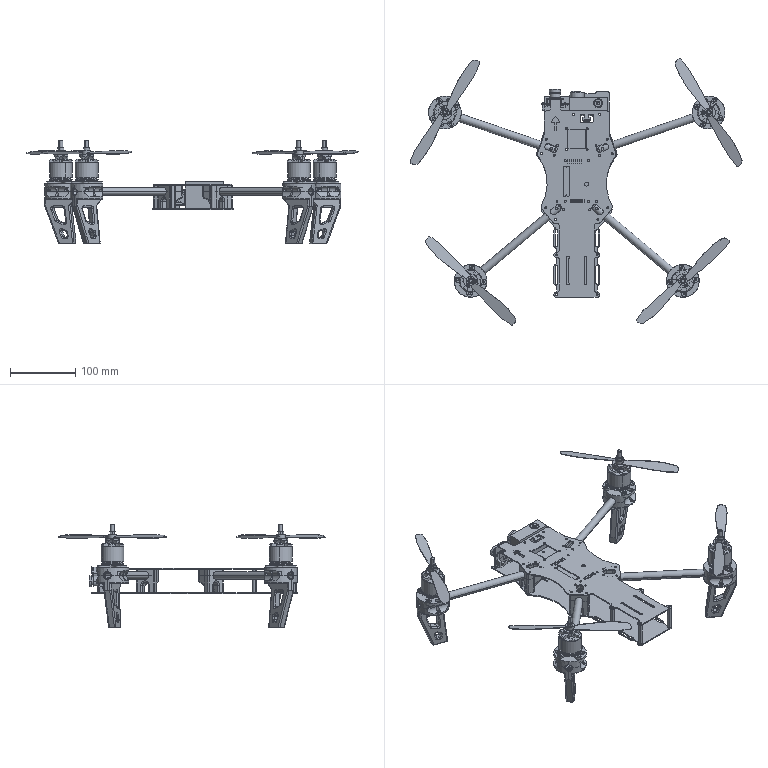Assembly | SolidWorks | mm | 49 component files | 49 solids | 2994 faces | box 508.26 x 408.35 x 158.75 mm | volume 593246 mm3 | cylinder 1614 | plane 994 | cone 152 | torus 112 | spline 76 | sphere 46 | commonest cylinder face diameters 4 x487 3 x165 8 x126 35 x76 2 x74 2.5 x64 16 x60 30 x48
Bill of materials:
Actuator | 1 |  | Thin rectangular plate with four corner holes. A stepped cylindrical body sticks out from one face, and several small rectangular blocks sit on the plate. Overall it resembles a board-mounted camera/lens module.
Adjuster | 4 |  | Short thick-walled cylindrical ring/bushing with a through bore. The outer edge on one end is chamfered or conical.
BaseConnectionPart | 4 |  | Flat, thin four-armed cross/X-shaped plate with rounded arm ends, generous fillets between arms, and a central hole. Each arm has two through-holes.
Camera | 1 |  | Rectangular block with a short cylindrical boss on one face. A shallow circular feature (ring or button outline) is on the top face.
ConnectingRod | 4 |  | Long straight hollow round tube with small radial cross-holes near each end.
Connector | 4 |  | Round disc base with a central upright cylindrical pin that has a chamfered tip. The disc has three through-holes with counterbores. The underside has large curved scallop cuts.
FanBlade | 4 |  | Two-bladed propeller-like part. A small cylindrical hub with a central through-bore has two long, thin, tapered and twisted blades sticking out in opposite directions.
LowerPartOfBracket | 4 |  | Short cylindrical puck-shaped hub. The top face has a small central hole, four radial slots and two counterbored holes. Large arched cutouts are around the lower side wall.
LowerPlate | 1 |  | Long, very thin, flat plate with a complex outline. It has a narrow waist with large concave curved sides and a central round hole. It also has many small holes, long slots, a T/key-shaped cutout, and paired slots along the edges of one end.
Motor | 4 |  | Cylindrical can-shaped body that resembles an outrunner-style motor. The top has spoked openings, a raised central boss, and small holes. Grooves and flange steps are near the bottom, and a short shaft sticks out at each end.
SupportPlate | 1 |  | Thin rectangular plate with a large central circular hole. There are small rectangular tabs on one short edge and matching notches on the opposite edge, with rounded corners.
UpperAndLowerPlateConnection | 4 |  | Thick, roughly square block with rounded corners and notched edges. It has a central elongated (obround) through-opening and four corner through-holes. A semicircular saddle cut runs across the underside.
UpperAndLowerPlateLowerConnectionPart | 4 |  | Block-shaped part with a semicircular channel running across its top face. Two flat flanges sit on either side of the channel, each with two through holes, so there are four holes in total. Underneath are two legs with an arched opening between them, which forms a channel at right angles to the top one.
UpperAndLowerPlateSupportColumn | 4 |  | Straight hollow cylinder (a tube or spacer) with a single concentric through bore and plain flat ends.
UpperPartOfBracket | 4 |  | Round flat-topped head on a tapered, slanted arm that gets narrower toward its free end. The top of the head has a wide central groove with a smaller hole in its floor. It also has two through holes, a small dome-shaped bump and several smaller grooves running parallel to the main one. The arm is a web with stiffening edges and two lightening cutouts with rounded corners: a large trapezoid and a smaller rounded slot.
UpperPlate | 1 |  | Thin flat plate, long and roughly symmetrical about its long axis. It has a wider middle section with curved, waisted sides and a narrower rectangular tail with two long parallel slots. A small tab sticks out from one end. The plate has many small round holes, four angled oblong slots, a square cutout, a long central slot, a single larger hole, two patches of tiny holes in a grid, an arrow-shaped cutout and a squared C-shaped cutout.
Mates:
1. concentric | LowerPlate-1 face at (-71.048, 32.401, 1000) dir (0, 0, 1) r 1.5 | UpperAndLowerPlateLowerConnectionPart-1 face at (-71.048, 32.401, 1027.6) dir (0, 0, -1) r 1.5
2. concentric | LowerPlate-1 face at (-63.432, 54.633, 1000) dir (0, 0, 1) r 1.5 | UpperAndLowerPlateLowerConnectionPart-1 face at (-63.432, 54.633, 1027.6) dir (0, 0, -1) r 1.5
3. coincident | LowerPlate-1 face at (14.261, -183.575, 1001.6) dir (0, 0, 1) | UpperAndLowerPlateLowerConnectionPart-1 face at (-50.912, 29.468, 1001.6) dir (0, 0, -1)
4. concentric | UpperAndLowerPlateLowerConnectionPart-1 face at (-71.048, 32.401, 1027.6) dir (0, 0, -1) r 1.5 | UpperAndLowerPlateConnection-1 face at (-71.048, 32.401, 1037.6) dir (0, 0, -1) r 1.5
5. concentric | UpperAndLowerPlateLowerConnectionPart-1 face at (-46.2, 44.766, 1027.6) dir (0, 0, -1) r 1.5 | UpperAndLowerPlateConnection-1 face at (-46.2, 44.766, 1037.6) dir (0, 0, -1) r 1.5
6. coincident | UpperAndLowerPlateLowerConnectionPart-1 face at (-50.912, 29.468, 1027.6) dir (0, 0, 1) | UpperAndLowerPlateConnection-1 face at (-59.183, 54.499, 1027.6) dir (0, 0, -1)
7. concentric | UpperAndLowerPlateLowerConnectionPart-1 face at (-44.535, 35.74, 1027.6) dir (-0.946, 0.3241, 0) r 6 | ConnectingRod-1 face at (-51.158, 38.008, 1027.6) dir (-0.946, 0.3241, 0) r 6
8. concentric | UpperAndLowerPlateConnection-1 face at (-70.078, 44.49, 1032.6) dir (0, 0, 1) r 2 | ConnectingRod-1 face at (-70.078, 44.49, 1033.6) dir (0, 0, -1) r 2
9. concentric | ConnectingRod-1 face at (-51.158, 38.008, 1027.6) dir (-0.946, 0.3241, 0) r 6 | LowerPartOfBracket-1 face at (-194.955, 87.266, 1027.6) dir (-0.946, 0.3241, 0) r 6
10. concentric | ConnectingRod-1 face at (-235.635, 101.2, 1033.6) dir (0, 0, -1) r 2 | LowerPartOfBracket-1 face at (-235.635, 101.2, 1032.6) dir (0, 0, 1) r 2
11. concentric | ConnectingRod-1 face at (-51.158, 38.008, 1027.6) dir (-0.946, 0.3241, 0) r 6 | UpperPartOfBracket-1 face at (-194.955, 87.266, 1027.6) dir (-0.946, 0.3241, 0) r 6
12. coincident | UpperPartOfBracket-1 face at (-218.606, 95.367, 1027.6) dir (0, 0, 1) | LowerPartOfBracket-1 face at (-218.606, 95.367, 1027.6) dir (0, 0, -1)
13. concentric | ConnectingRod-1 face at (-235.635, 101.2, 1033.6) dir (0, 0, -1) r 2 | UpperPartOfBracket-1 face at (-235.635, 101.2, 1022.6) dir (0, 0, -1) r 2
14. width | BaseConnectionPart-1 face at (-216.847, 91.775, 1042.6) dir (0.4398, -0.8981, 0) | BaseConnectionPart-1 face at (-220.365, 98.96, 1042.6) dir (-0.4398, 0.8981, 0) | LowerPartOfBracket-1 face at (-224.911, 90.053, 1026.263) dir (-0.4398, 0.8981, 0) | LowerPartOfBracket-1 face at (-226.67, 93.645, 1026.263) dir (0.4398, -0.8981, 0)
15. width | BaseConnectionPart-1 face at (-222.198, 93.608, 1042.6) dir (-0.8981, -0.4398, 0) | BaseConnectionPart-1 face at (-215.014, 97.126, 1042.6) dir (0.8981, 0.4398, 0) | LowerPartOfBracket-1 face at (-223.921, 101.672, 1026.263) dir (0.8981, 0.4398, 0) | LowerPartOfBracket-1 face at (-220.328, 103.431, 1026.263) dir (-0.8981, -0.4398, 0)
16. coincident | LowerPartOfBracket-1 face at (-218.606, 95.367, 1039.6) dir (0, 0, 1) | BaseConnectionPart-1 face at (-218.606, 95.367, 1039.6) dir (0, 0, -1)
17. concentric | BaseConnectionPart-1 face at (-213.108, 84.141, 1039.6) dir (0, 0, -1) r 1.7 | Motor-1 face at (-213.108, 84.141, 1042.6) dir (0, 0, -1) r 1.25
18. concentric | BaseConnectionPart-1 face at (-210.074, 99.545, 1039.6) dir (0, 0, -1) r 1.7 | Motor-1 face at (-210.074, 99.545, 1042.6) dir (0, 0, -1) r 1.25
19. concentric | BaseConnectionPart-1 face at (-218.606, 95.367, 1039.6) dir (0, 0, 1) r 2.25 | Motor-1 face at (-218.606, 95.367, 1078.15) dir (0, 0, 1) r 2
20. coincident | BaseConnectionPart-1 face at (-218.606, 95.367, 1042.6) dir (0, 0, 1) | Motor-1 face at (-220.402, 94.488, 1042.6) dir (0, 0, -1)
21. concentric | Motor-1 face at (-222.79, 89.143, 1069.85) dir (0, 0, 1) r 1 | Connector-1 face at (-222.79, 89.143, 1084.35) dir (0, 0, 1) r 1.45
22. concentric | Motor-1 face at (-211.123, 94.856, 1069.85) dir (0, 0, 1) r 1 | Connector-1 face at (-211.123, 94.856, 1084.35) dir (0, 0, 1) r 1.45
23. coincident | Motor-1 face at (-223.096, 93.168, 1078.35) dir (0, 0, 1) | Connector-1 face at (-218.606, 95.367, 1078.35) dir (0, 0, -1)
24. concentric | Connector-1 face at (-218.606, 95.367, 1076.35) dir (0, 0, -1) r 3 | FanBlade-1 face at (-218.606, 95.367, 1075.65) dir (0, 0, 1) r 3.25
25. coincident | Connector-1 face at (-209.892, 89.509, 1084.35) dir (0, 0, 1) | FanBlade-1 face at (-218.606, 95.367, 1084.35) dir (0, 0, -1)
26. coincident | LowerPlate-1 face at (14.261, -183.575, 1001.6) dir (0, 0, 1) | SupportPlate-1 face at (-47.616, 116.675, 1001.6) dir (0, 0, -1)
27. parallel | LowerPlate-1 face at (33.261, 120.425, 1001.6) dir (0, 1, 0) | SupportPlate-1 face at (-50.116, 116.675, 1018.85) dir (0, 1, 0)
28. parallel | LowerPlate-1 face at (-66.739, 64.711, 1001.6) dir (-1, 0, 0) | SupportPlate-1 face at (-62.616, 116.675, 1000.1) dir (-1, 0, 0)
29. coincident | LowerPlate-1 face at (-61.077, 116.675, 1000) dir (0, -1, 0) | SupportPlate-1 face at (-50.116, 116.675, 1018.85) dir (0, 1, 0)
30. lock | LowerPlate-1 reference at (0, 0, 0) dir (1, 0, 0) | SupportPlate-1 reference at (0, 0, 0) dir (1, 0, 0)
31. concentric | SupportPlate-1 face at (-50.116, 116.675, 1018.85) dir (0, -1, 0) r 8 | Actuator-1 face at (-50.116, 108.825, 1018.85) dir (0, -1, 0) r 8
32. coincident | SupportPlate-1 face at (-50.116, 115.175, 1018.85) dir (0, -1, 0) | Actuator-1 face at (-50.116, 115.175, 1018.85) dir (0, 1, 0)
33. parallel | SupportPlate-1 face at (-54.616, 116.675, 1037.6) dir (0, 0, 1) | Actuator-1 face at (-70.116, 107.325, 1031.35) dir (0, 0, 1)
34. coincident | LowerPlate-1 face at (14.261, -183.575, 1001.6) dir (0, 0, 1) | Camera-1 face at (30.917, 118.685, 1001.6) dir (0, 0, -1)
35. parallel | LowerPlate-1 face at (-51.739, -165.575, 1001.6) dir (-1, 0, 0) | UpperPlate-3 face at (-43.739, -176.647, 1039.2) dir (-1, 0, 0)
36. concentric | LowerPlate-1 face at (-47.739, -183.575, 1000) dir (0, 0, 1) r 1.5 | UpperPlate-3 face at (-47.739, -183.575, 1037.6) dir (0, 0, 1) r 1.5
37. concentric | UpperAndLowerPlateSupportColumn-1 face at (-47.739, -122.575, 1037.6) dir (0, 0, -1) r 1.5 | UpperPlate-3 face at (-47.739, -122.575, 1037.6) dir (0, 0, 1) r 1.5
38. coincident | LowerPlate-1 face at (14.261, -183.575, 1001.6) dir (0, 0, 1) | UpperAndLowerPlateSupportColumn-1 face at (-47.739, -122.575, 1001.6) dir (0, 0, -1)
39. concentric | UpperPlate-3 face at (-47.739, -183.575, 1037.6) dir (0, 0, 1) r 1.5 | UpperAndLowerPlateSupportColumn-2 face at (-47.739, -183.575, 1037.6) dir (0, 0, -1) r 1.5
40. coincident | LowerPlate-1 face at (14.261, -183.575, 1001.6) dir (0, 0, 1) | UpperAndLowerPlateSupportColumn-2 face at (-47.739, -183.575, 1001.6) dir (0, 0, -1)
41. concentric | UpperPlate-3 face at (14.261, -183.575, 1037.6) dir (0, 0, 1) r 1.5 | UpperAndLowerPlateSupportColumn-3 face at (14.261, -183.575, 1037.6) dir (0, 0, -1) r 1.5
42. coincident | LowerPlate-1 face at (14.261, -183.575, 1001.6) dir (0, 0, 1) | UpperAndLowerPlateSupportColumn-3 face at (14.261, -183.575, 1001.6) dir (0, 0, -1)
43. concentric | UpperPlate-3 face at (14.261, -122.575, 1037.6) dir (0, 0, 1) r 1.5 | UpperAndLowerPlateSupportColumn-4 face at (14.261, -122.575, 1037.6) dir (0, 0, -1) r 1.5
44. coincident | LowerPlate-1 face at (14.261, -183.575, 1001.6) dir (0, 0, 1) | UpperAndLowerPlateSupportColumn-4 face at (14.261, -122.575, 1001.6) dir (0, 0, -1)
45. coincident | UpperPlate-3 face at (14.261, -183.575, 1037.6) dir (0, 0, -1) | UpperAndLowerPlateSupportColumn-3 face at (14.261, -183.575, 1037.6) dir (0, 0, 1)
46. lock | LowerPlate-1 reference at (0, 0, 0) dir (1, 0, 0) | UpperAndLowerPlateSupportColumn-4 reference at (0, 0, 0) dir (1, 0, 0)
47. lock | LowerPlate-1 reference at (0, 0, 0) dir (1, 0, 0) | UpperAndLowerPlateSupportColumn-3 reference at (0, 0, 0) dir (1, 0, 0)
48. lock | LowerPlate-1 reference at (0, 0, 0) dir (1, 0, 0) | UpperAndLowerPlateSupportColumn-2 reference at (0, 0, 0) dir (1, 0, 0)
49. lock | LowerPlate-1 reference at (0, 0, 0) dir (1, 0, 0) | UpperAndLowerPlateSupportColumn-1 reference at (0, 0, 0) dir (1, 0, 0)
50. concentric | LowerPlate-1 face at (-49.097, -68.575, 1000) dir (0, 0, 1) r 1.5 | UpperAndLowerPlateLowerConnectionPart-2 face at (-49.097, -68.575, 1027.6) dir (0, 0, -1) r 1.5
51. concentric | LowerPlate-1 face at (-64.203, -50.573, 1000) dir (0, 0, 1) r 1.5 | UpperAndLowerPlateLowerConnectionPart-2 face at (-64.203, -50.573, 1027.6) dir (0, 0, -1) r 1.5
52. coincident | LowerPlate-1 face at (14.261, -183.575, 1001.6) dir (0, 0, 1) | UpperAndLowerPlateLowerConnectionPart-2 face at (-36.187, -52.847, 1001.6) dir (0, 0, -1)
53. concentric | UpperAndLowerPlateLowerConnectionPart-2 face at (-64.203, -50.573, 1027.6) dir (0, 0, -1) r 1.5 | UpperAndLowerPlateConnection-2 face at (-64.203, -50.573, 1037.6) dir (0, 0, -1) r 1.5
54. concentric | UpperAndLowerPlateLowerConnectionPart-2 face at (-49.097, -68.575, 1027.6) dir (0, 0, -1) r 1.5 | UpperAndLowerPlateConnection-2 face at (-49.097, -68.575, 1037.6) dir (0, 0, -1) r 1.5
55. concentric | UpperAndLowerPlateLowerConnectionPart-2 face at (-46.854, -40.912, 1027.6) dir (0, 0, -1) r 1.5 | UpperAndLowerPlateConnection-2 face at (-46.854, -40.912, 1037.6) dir (0, 0, -1) r 1.5
56. coincident | UpperAndLowerPlateLowerConnectionPart-2 face at (-36.187, -52.847, 1027.6) dir (0, 0, 1) | UpperAndLowerPlateConnection-2 face at (-61.893, -47.004, 1027.6) dir (0, 0, -1)
57. concentric | UpperAndLowerPlateLowerConnectionPart-2 face at (-38.265, -44.147, 1027.6) dir (-0.766, -0.6428, 0) r 6 | ConnectingRod-2 face at (-43.627, -48.647, 1027.6) dir (-0.766, -0.6428, 0) r 6
58. concentric | UpperAndLowerPlateConnection-2 face at (-58.948, -61.503, 1032.6) dir (0, 0, 1) r 2 | ConnectingRod-2 face at (-58.948, -61.503, 1033.6) dir (0, 0, -1) r 2
59. concentric | ConnectingRod-2 face at (-43.627, -48.647, 1027.6) dir (-0.766, -0.6428, 0) r 6 | UpperPartOfBracket-2 face at (-160.066, -146.351, 1027.6) dir (-0.766, -0.6428, 0) r 6
60. concentric | ConnectingRod-2 face at (-193.006, -173.991, 1033.6) dir (0, 0, -1) r 2 | UpperPartOfBracket-2 face at (-193.006, -173.991, 1022.6) dir (0, 0, -1) r 2
61. concentric | ConnectingRod-2 face at (-43.627, -48.647, 1027.6) dir (-0.766, -0.6428, 0) r 6 | LowerPartOfBracket-2 face at (-160.066, -146.351, 1027.6) dir (-0.766, -0.6428, 0) r 6
62. concentric | ConnectingRod-2 face at (-193.006, -173.991, 1033.6) dir (0, 0, -1) r 2 | LowerPartOfBracket-2 face at (-193.006, -173.991, 1032.6) dir (0, 0, 1) r 2
63. width | BaseConnectionPart-2 face at (-179.566, -166.405, 1042.6) dir (-0.08716, -0.9962, 0) | BaseConnectionPart-2 face at (-178.868, -158.436, 1042.6) dir (0.08716, 0.9962, 0) | LowerPartOfBracket-2 face at (-171.073, -161.125, 1026.263) dir (-0.08716, -0.9962, 0) | LowerPartOfBracket-2 face at (-171.422, -165.11, 1026.263) dir (0.08716, 0.9962, 0)
64. width | BaseConnectionPart-2 face at (-179.566, -166.405, 1042.6) dir (-0.08716, -0.9962, 0) | BaseConnectionPart-2 face at (-178.868, -158.436, 1042.6) dir (0.08716, 0.9962, 0) | LowerPartOfBracket-2 face at (-187.361, -163.716, 1026.263) dir (0.08716, 0.9962, 0) | LowerPartOfBracket-2 face at (-187.012, -159.731, 1026.263) dir (-0.08716, -0.9962, 0)
65. width | BaseConnectionPart-2 face at (-183.202, -162.072, 1042.6) dir (-0.9962, 0.08716, 0) | BaseConnectionPart-2 face at (-175.232, -162.769, 1042.6) dir (0.9962, -0.08716, 0) | LowerPartOfBracket-2 face at (-181.907, -170.216, 1026.263) dir (0.9962, -0.08716, 0) | LowerPartOfBracket-2 face at (-177.922, -170.564, 1026.263) dir (-0.9962, 0.08716, 0)
66. coincident | LowerPartOfBracket-2 face at (-179.217, -162.42, 1039.6) dir (0, 0, 1) | BaseConnectionPart-2 face at (-179.217, -162.42, 1039.6) dir (0, 0, -1)
67. concentric | BaseConnectionPart-2 face at (-179.217, -162.42, 1039.6) dir (0, 0, 1) r 2.25 | Motor-2 face at (-179.217, -162.42, 1078.15) dir (0, 0, 1) r 2
68. concentric | BaseConnectionPart-2 face at (-191.67, -161.331, 1039.6) dir (0, 0, -1) r 1.7 | Motor-2 face at (-191.67, -161.331, 1042.6) dir (0, 0, -1) r 1.25
69. concentric | BaseConnectionPart-2 face at (-180.045, -171.884, 1039.6) dir (0, 0, -1) r 1.7 | Motor-2 face at (-180.045, -171.884, 1042.6) dir (0, 0, -1) r 1.25
70. coincident | BaseConnectionPart-2 face at (-179.217, -162.42, 1042.6) dir (0, 0, 1) | Motor-2 face at (-179.043, -160.428, 1042.6) dir (0, 0, -1)
71. concentric | Motor-2 face at (-183.519, -168.564, 1069.85) dir (0, 0, 1) r 1 | Connector-2 face at (-183.519, -168.564, 1084.35) dir (0, 0, 1) r 1.45
72. concentric | Motor-2 face at (-182.387, -155.623, 1069.85) dir (0, 0, 1) r 1 | Connector-2 face at (-182.387, -155.623, 1084.35) dir (0, 0, 1) r 1.45
73. coincident | Motor-2 face at (-178.781, -157.439, 1078.35) dir (0, 0, 1) | Connector-2 face at (-179.217, -162.42, 1078.35) dir (0, 0, -1)
74. concentric | Connector-2 face at (-179.217, -162.42, 1076.35) dir (0, 0, -1) r 3 | FanBlade-2 face at (-179.217, -162.42, 1075.65) dir (0, 0, 1) r 3.25
75. coincident | Connector-2 face at (-170.616, -168.443, 1084.35) dir (0, 0, 1) | FanBlade-2 face at (-179.217, -162.42, 1084.35) dir (0, 0, -1)
76. concentric | Connector-1 face at (-218.606, 95.367, 1076.35) dir (0, 0, -1) r 3 | Adjuster-1 face at (-218.606, 95.367, 1095.85) dir (0, 0, -1) r 3
77. coincident | FanBlade-1 face at (-218.606, 95.367, 1090.85) dir (0, 0, 1) | Adjuster-1 face at (-218.606, 95.367, 1090.85) dir (0, 0, -1)
78. concentric | Connector-2 face at (-179.217, -162.42, 1076.35) dir (0, 0, -1) r 3 | Adjuster-2 face at (-179.217, -162.42, 1095.85) dir (0, 0, -1) r 3
79. coincident | FanBlade-2 face at (-179.217, -162.42, 1090.85) dir (0, 0, 1) | Adjuster-2 face at (-179.217, -162.42, 1090.85) dir (0, 0, -1)
80. lock | Motor-1 reference at (0, 0, 0) dir (1, 0, 0) | Adjuster-1 reference at (0, 0, 0) dir (1, 0, 0)
81. parallel | LowerPlate-1 face at (16.261, 127.925, 1000) dir (0, 1, 0) | Camera-1 face at (-16.083, 118.685, 1030.6) dir (0, 1, 0)
82. coincident | Camera-1 edge at (-28.083, 97.685, 1042.6) dir (1, 0, 0) | UpperPlate-3 face at (33.261, 97.685, 1039.2) dir (0, 1, 0)
83. lock | Camera-1 reference at (0, 0, 0) dir (1, 0, 0) | UpperPlate-3 reference at (0, 0, 0) dir (1, 0, 0)